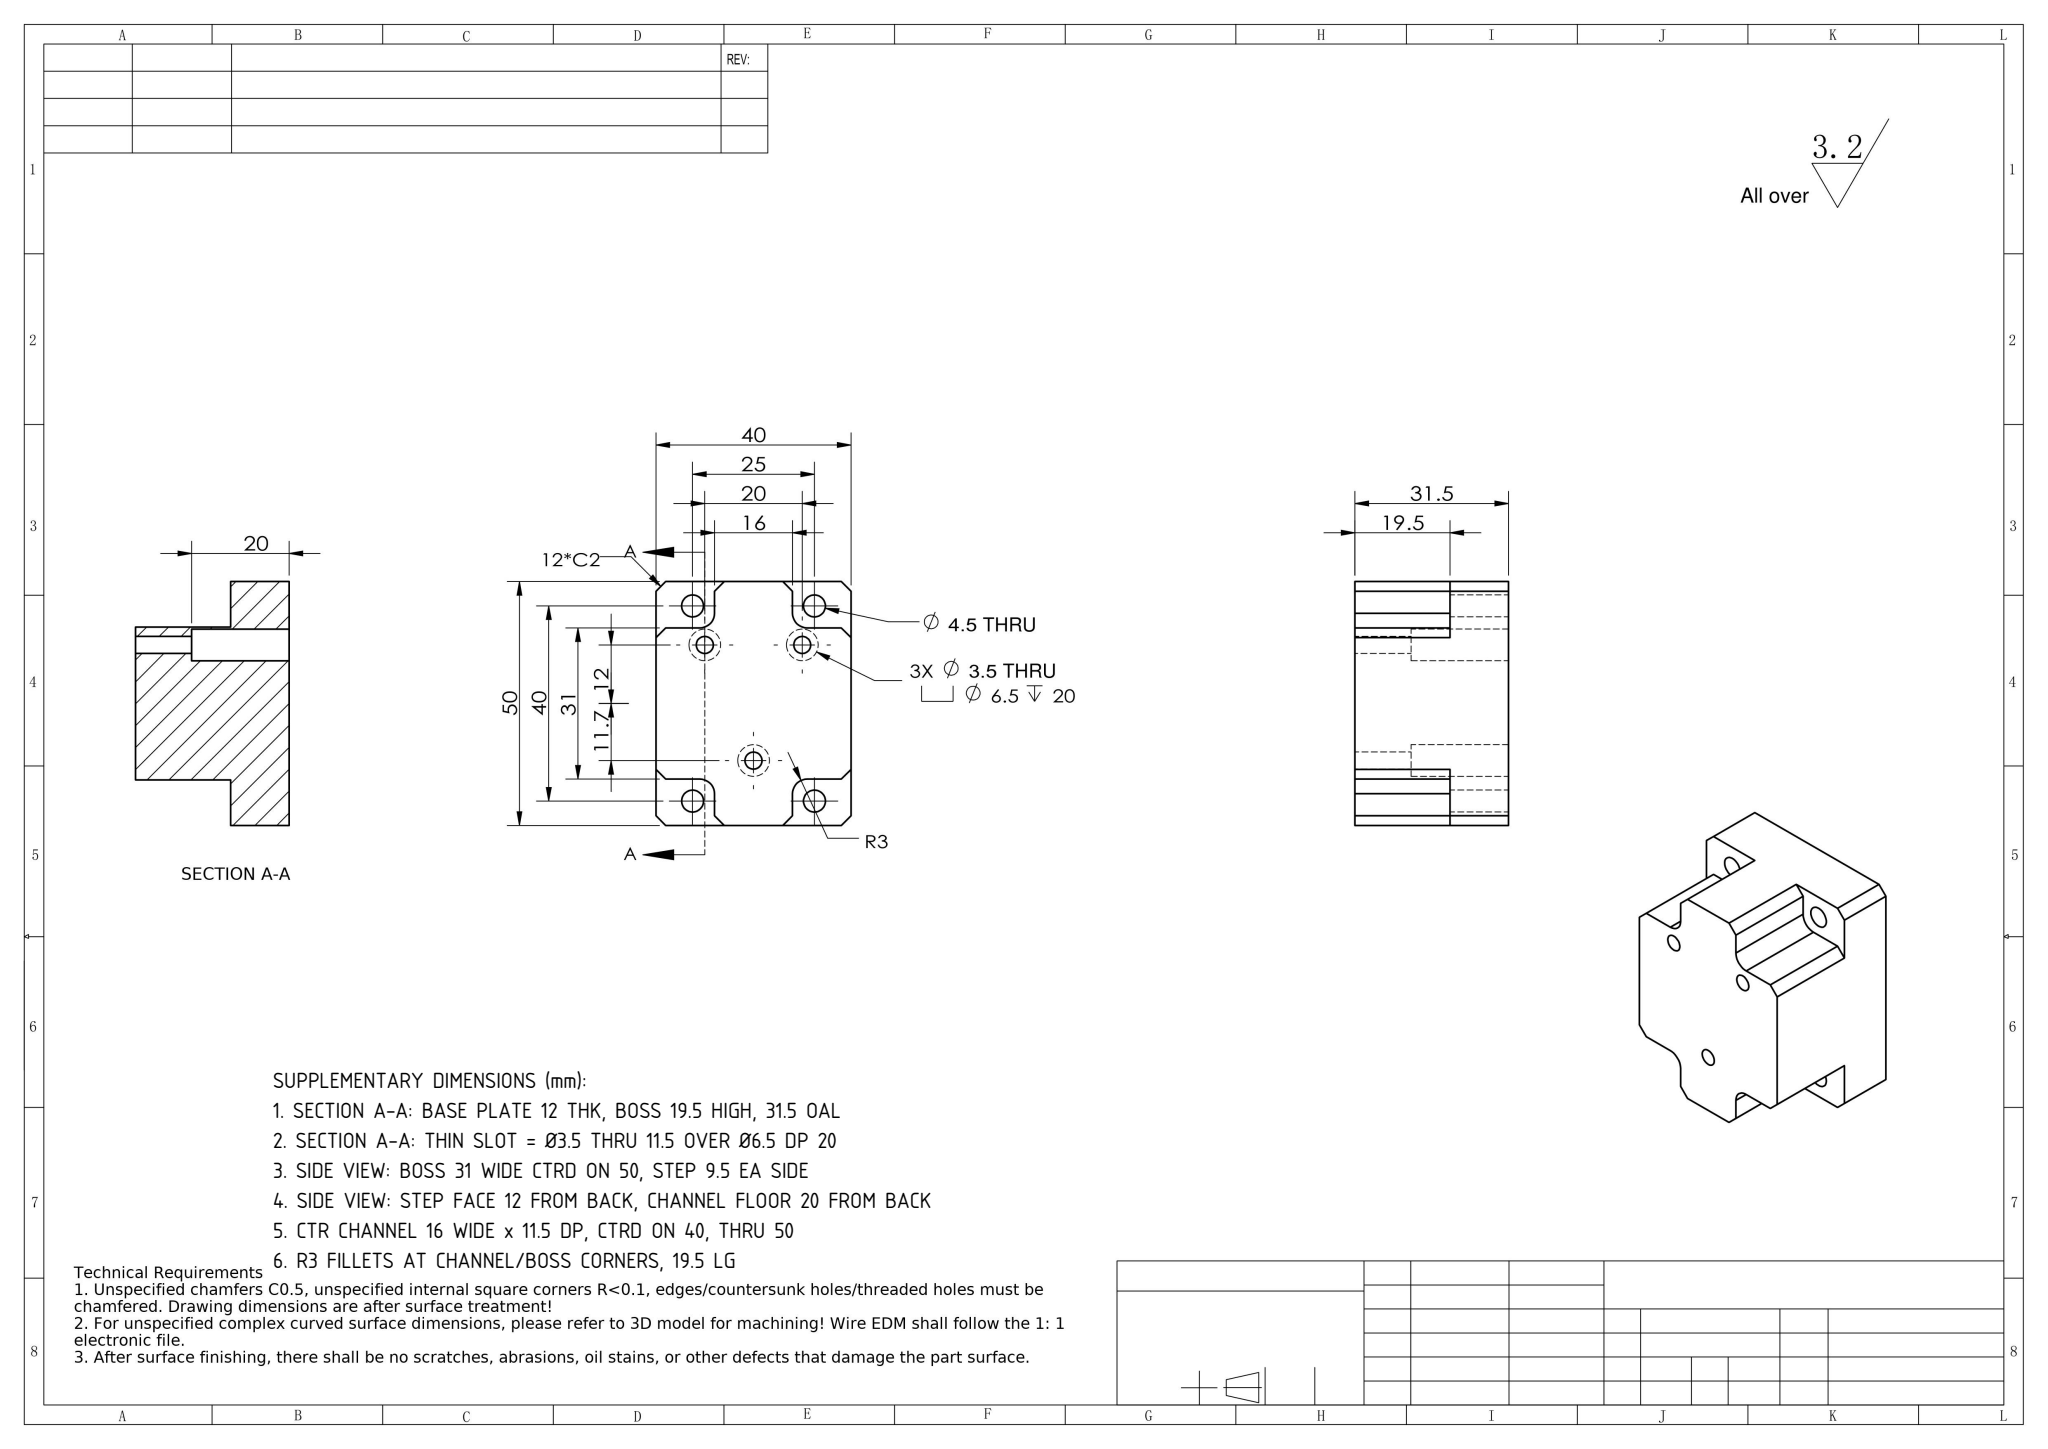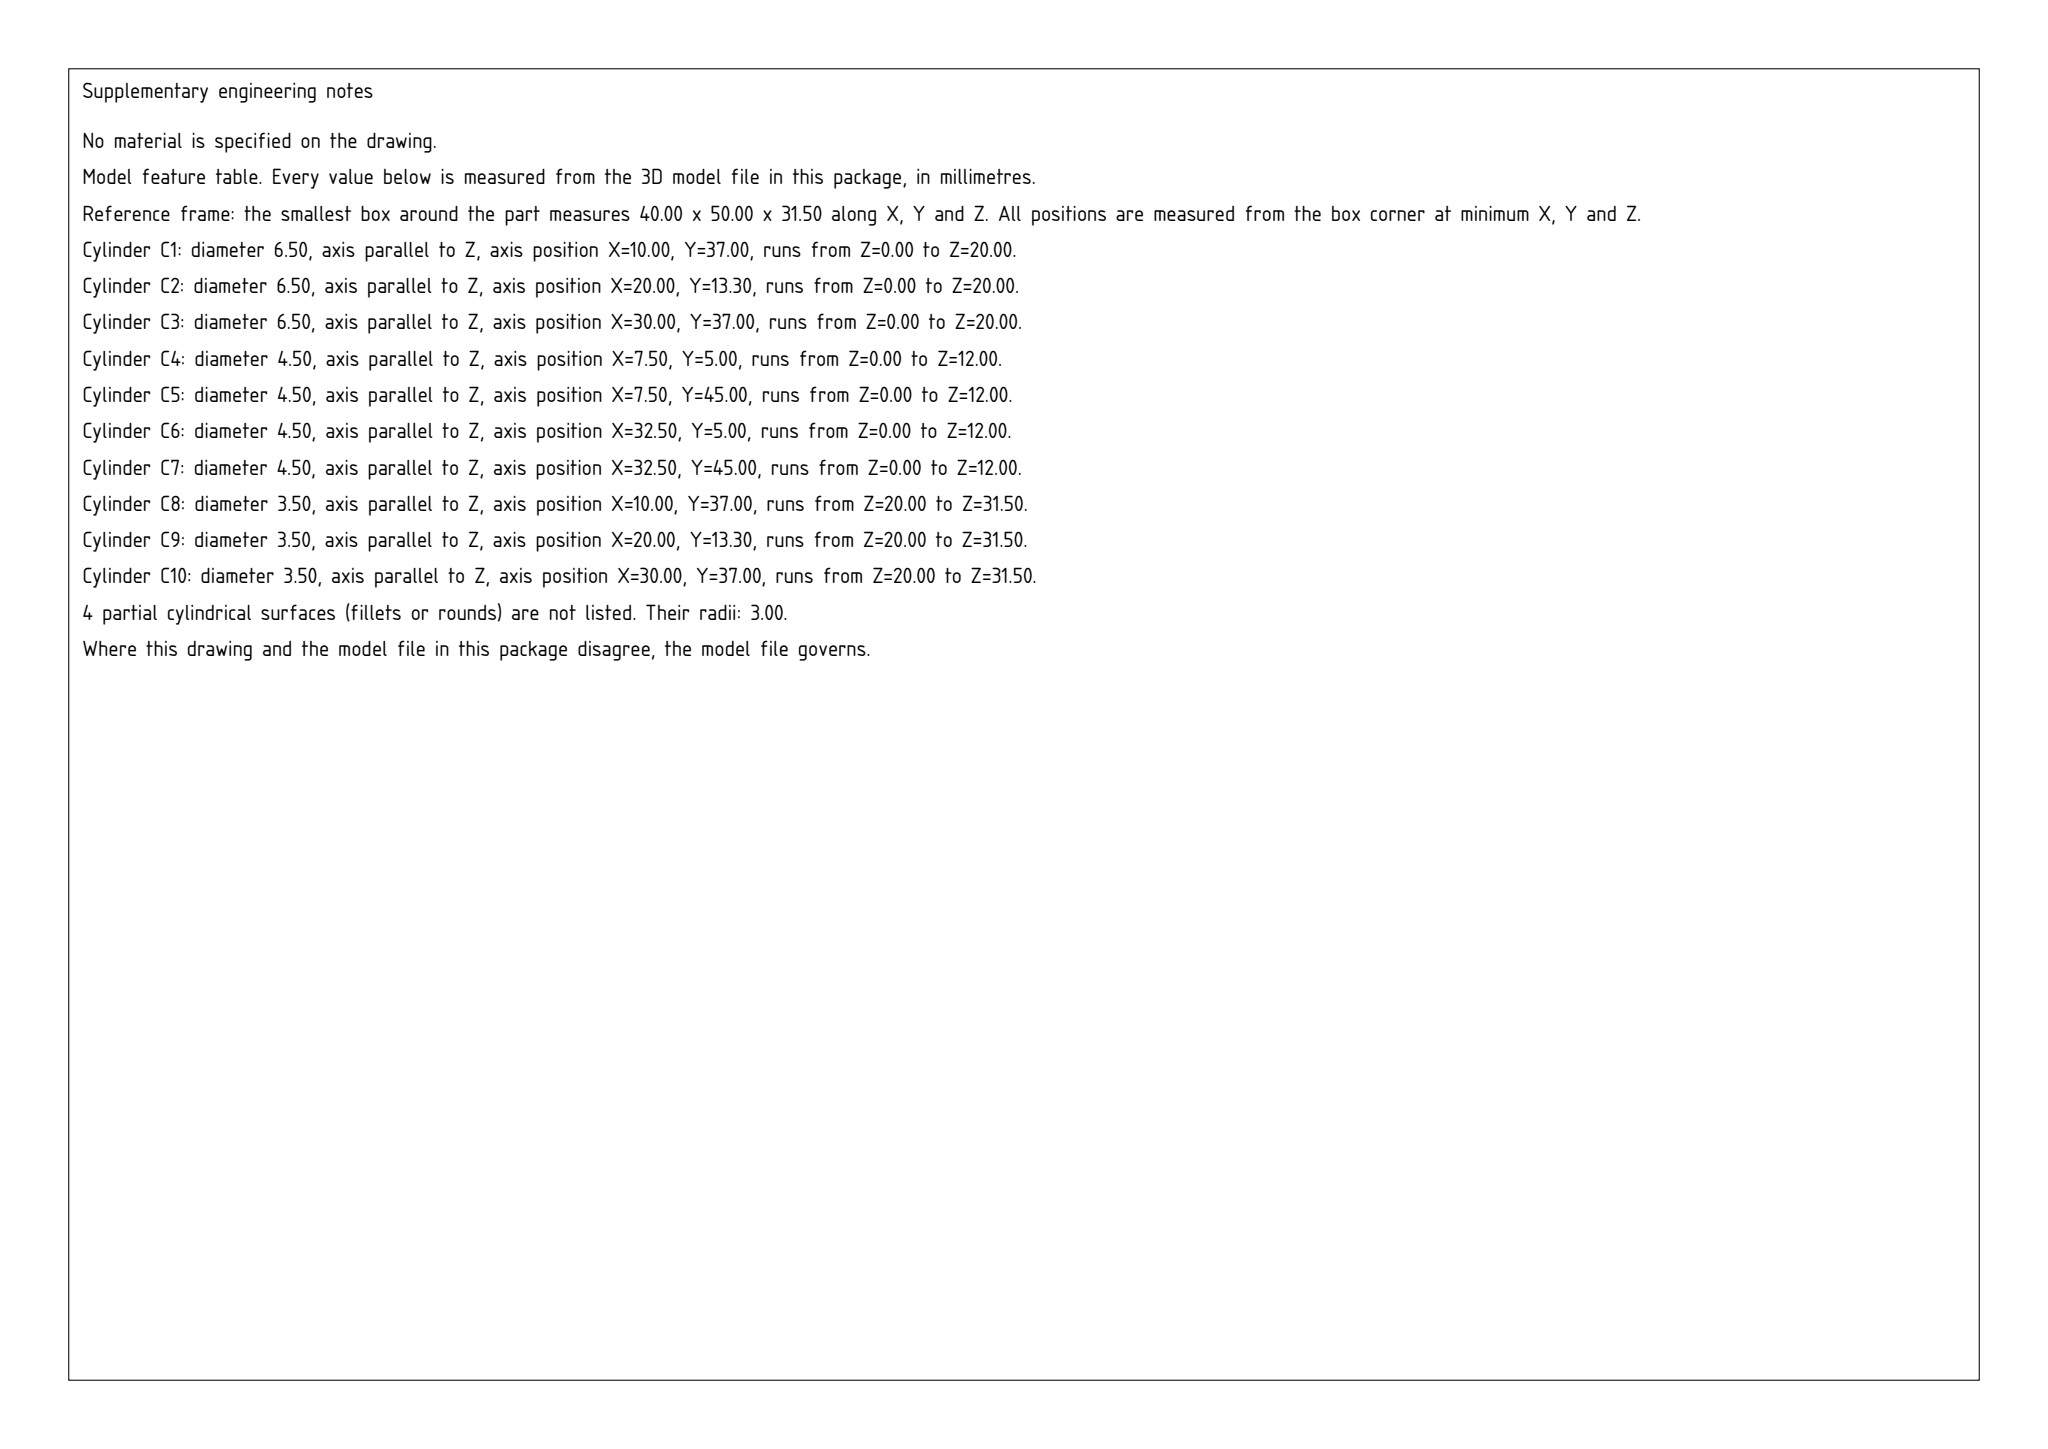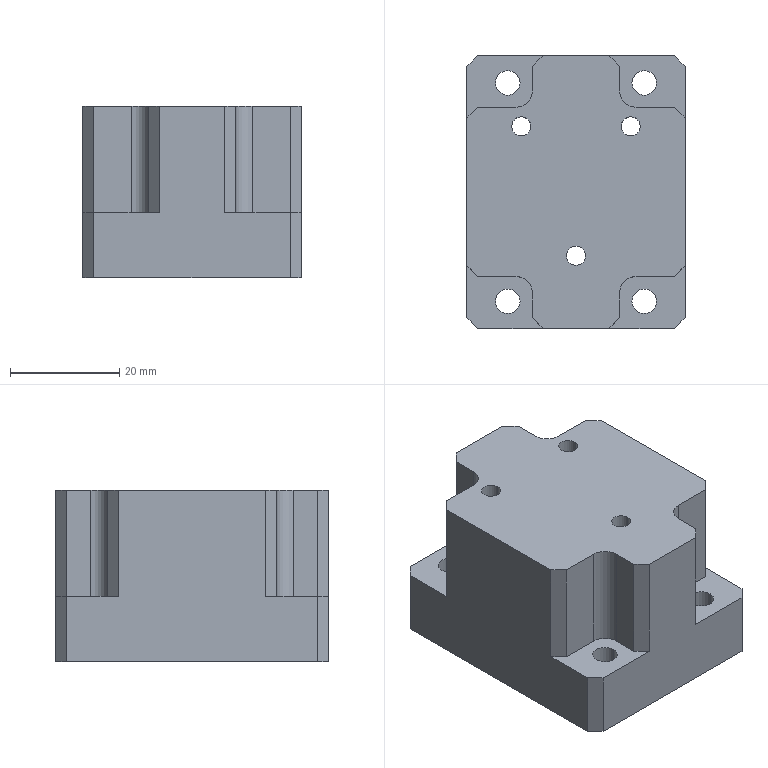Part | SolidWorks | mm | 1 solid | 57 faces | box 40 x 50 x 31.5 mm | volume 50764 mm3 | plane 33 | cylinder 24 | commonest cylinder face diameters 4.5 x8 6.5 x6 3.5 x6 6 x4
build123d program:
from build123d import *

# Parameters (mm, degrees)
SKETCH1_W            = 40
SKETCH1_H            = 50
BOSS_EXTRUDE1_DEPTH  = 31.5
SKETCH2_W            = 12
SKETCH2_H            = 9.5
CUT_EXTRUDE1_DEPTH   = 19.5
FILLET1_R            = 3
CHAMFER1_SIZE        = 2
M4_CLEARANCE_HOLE1_D = 4.5
CHAMFER2_SIZE        = 2
HOLE1_D              = 3.5
HOLE1_CBORE_D        = 6.5
HOLE1_CBORE_DEPTH    = 20


with BuildPart() as part:
    # Sketch1 → Boss-Extrude1 (new body)
    with BuildSketch(Plane.XY):
        Rectangle(SKETCH1_W, SKETCH1_H)
    extrude(amount=BOSS_EXTRUDE1_DEPTH)

    # Sketch2 → Cut-Extrude1 (cut)
    with BuildSketch(Plane.XY.offset(31.5)):
        with Locations((-14, 20.25)):
            Rectangle(SKETCH2_W, SKETCH2_H)
        with Locations((14, 20.25)):
            Rectangle(SKETCH2_W, SKETCH2_H)
        with Locations((14, -20.25)):
            Rectangle(SKETCH2_W, SKETCH2_H)
        with Locations((-14, -20.25)):
            Rectangle(SKETCH2_W, SKETCH2_H)
    extrude(amount=-CUT_EXTRUDE1_DEPTH, mode=Mode.SUBTRACT)

    # Fillet1
    fillet1_edges = [part.edges().sort_by_distance(p)[0] for p in [
        (-8, 15.5, 21.75),
        (8, 15.5, 21.75),
        (8, -15.5, 21.75),
        (-8, -15.5, 21.75),
    ]]
    fillet(fillet1_edges, radius=FILLET1_R)

    # Chamfer1
    chamfer1_edges = [part.edges().sort_by_distance(p)[0] for p in [
        (-20, 15.5, 21.75),
        (-8, 25, 21.75),
        (20, 15.5, 21.75),
        (8, 25, 21.75),
        (20, -15.5, 21.75),
        (8, -25, 21.75),
        (-20, -15.5, 21.75),
        (-8, -25, 21.75),
    ]]
    chamfer(chamfer1_edges, length=CHAMFER1_SIZE)

    # M4 Clearance Hole1 (through all)
    with Locations(Plane(origin=(0, 0, 0), x_dir=(-1, 0, 0), z_dir=(0, 0, -1))):
        with Locations((-12.5, 20), (12.5, 20), (-12.5, -20), (12.5, -20)):
            Hole(M4_CLEARANCE_HOLE1_D / 2)

    # Chamfer2
    chamfer2_edges = [part.edges().sort_by_distance(p)[0] for p in [
        (-20, 25, 6),
        (20, -25, 6),
        (-20, -25, 6),
        (20, 25, 6),
    ]]
    chamfer(chamfer2_edges, length=CHAMFER2_SIZE)

    # Hole1 (through all)
    with Locations(Plane(origin=(0, 0, 0), x_dir=(-1, 0, 0), z_dir=(0, 0, -1))):
        with Locations((10, 12), (-10, 12), (0, -11.7)):
            CounterBoreHole(HOLE1_D / 2, HOLE1_CBORE_D / 2, HOLE1_CBORE_DEPTH)


solid = part.part